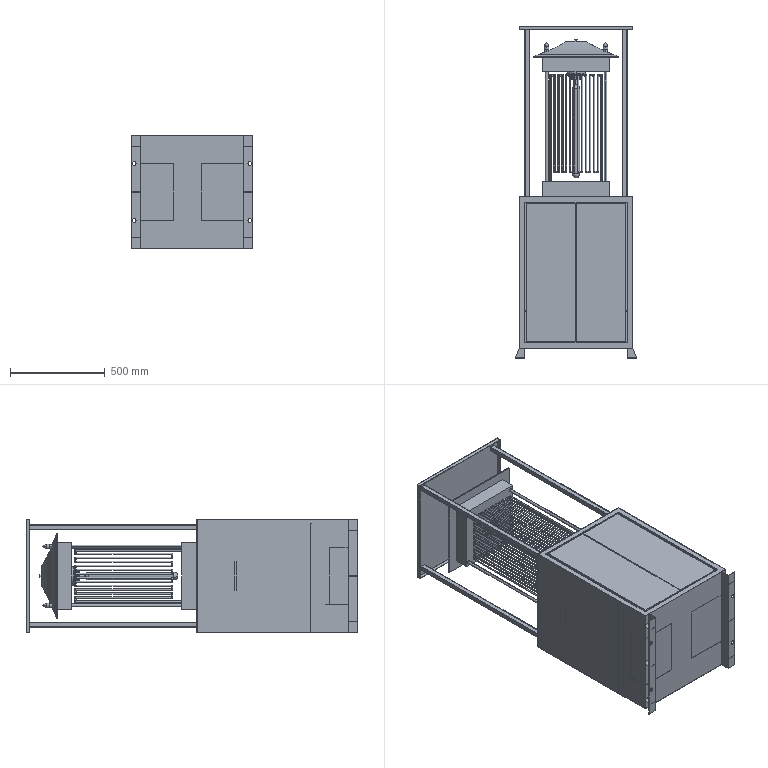Assembly | SolidWorks | mm | 47 component files | 47 solids | 2764 faces | box 640 x 1750 x 600 mm | volume 31033976 mm3 | cylinder 1488 | plane 1206 | torus 40 | spline 26 | sphere 4 | commonest cylinder face diameters 1 x1001 7 x210 5 x88 2.8 x31 20 x28 15 x26 6 x16 8 x14
Bill of materials:
AwningSupportRod | 4 |  | Long straight hollow tube with a square cross-section and thin walls.
AwningTopPlate | 1 |  | Thin, flat, square plate with no visible features.
Box | 1 |  | Rectangular box made of thin walls with an open top. It has flanges on the vertical front edges with small holes, a rectangular cutout in one wall, small triangular tabs along one edge, and angled foot-like tabs at the bottom.
Brush | 3 |  | Long strip with a raised rectangular rib along one edge and a row of many fine, closely spaced bristles or teeth along the other edge, like a comb.
CabinetDoor | 2 |  | Thin rectangular flat plate with small holes near the ends of its long edges and small square openings visible in the end edge view.
Camera | 1 |  | Square block body with a stepped cylindrical boss and a small side pin on one face. A rectangular arm extends from the block and ends in a flat circular disc.
CameraFillLightBracketTable | 1 |  | Rectangular plate of moderate thickness with a small chamfer or bevel along one edge.
FillLight | 1 |  | Flat annular ring with a thin rectangular tab extending outward from its outer edge.
Funnel | 1 |  | Square pyramid-shaped funnel or horn with a square rim at the wide end. It narrows to a rectangular throat block, which carries a short cylindrical tube stub and an angled side tab.
InfraredProcessingChamber | 1 |  | Thin sheet bent into a U or C-channel shape: two parallel flat faces joined by one back face. One face has a square cutout.
InsectCollectionBox | 1 |  | Solid rectangular block with no visible holes or features.
InsectCollectionPlatform | 1 |  | Thin flat plate with a large rectangular notch cut in from one edge, one round hole, two small square holes, and small raised tab or lug features near one edge.
BracketRod | 4 |  | Straight, slender solid cylindrical rod with flat ends.
ElectricNet | 1 |  | Continuous round-section tube or wire bent into a multi-pass serpentine with many parallel straight runs joined by tight U-bends, filling a rectangular box-shaped envelope, with two straight free ends.
InsectTrapLampBase | 1 |  | Square plate of moderate thickness with one large central circular through hole.
InsectTrapLampTop | 1 |  | Composite square body: a thin square flange plate with a rectangular block on one side. The block face carries four small corner holes and a central stepped concentric circular boss with a small central hole. The opposite side of the flange has a flared, curved-profile taper ending in a smaller flat face with protruding cylindrical pins.
LampTube | 1 |  | Elongated capsule-shaped cylindrical body with hemispherical or rounded ends, and a much thinner coaxial rod or wire extending from one end.
LeftPlatform | 1 |  | Thin square sheet or plate with a narrow short lip bent at about 90 degrees along one edge, giving a shallow L-shaped section.
Pin | 4 |  | Solid flanged cylinder: a cylindrical body standing on a larger-diameter thin circular flange whose outer bottom edge is rounded.
PushRod | 1 |  | Straight, slender solid cylindrical rod with flat ends.
PushRodCylinder | 1 |  | Thick-walled cylindrical sleeve, longer than its diameter, with a small coaxial bore.
PushRodFixingRing | 2 |  | Short thin-walled ring or band with a large central opening, with one outer circumferential edge rounded.
SlideRailSupport | 2 |  | Rectangular block with one rounded long edge and two round holes on perpendicular axes: one in the top face and one in a side face.
SlideRod | 2 |  | Very slender straight solid cylindrical rod or wire with flat ends.
SlideTablePlatform | 1 |  | Thin rectangular plate with raised rectangular pads/blocks at both ends of one face, positioned near the corners, with small holes through the blocks and edge.
TopCover | 4 |  | Axisymmetric cap: a hollow cylindrical sleeve that steps down into a closed, domed end with a turned stepped/bulbous profile.
WaterCollectionBox | 1 |  | Plain solid rectangular block (cuboid) with no visible features.
WaterPipe | 1 |  | Hollow round tube bent along a 3D path with several bends, open at both ends.
WireBox | 1 |  | Rectangular box-shaped enclosure or body with chamfered edges, with several rectangular openings on one narrow end face.
Mates:
1. coincident | Box-1 face at (298.5, 800, -300) dir (-1, 0, 0) | InfraredProcessingChamber-1 face at (298.5, 270, 0) dir (1, 0, 0)
2. coincident | Box-1 plane at (0, 0, 0) dir (0, 0, 1) | InfraredProcessingChamber-1 plane at (175, 270, 0) dir (0, 0, 1)
3. coincident | Box-1 face at (0, 1.5, 0) dir (0, 1, 0) | InsectCollectionBox-1 face at (173.5, 1.5, 0) dir (0, -1, 0)
4. coincident | Box-1 face at (298.5, 800, -300) dir (-1, 0, 0) | InsectCollectionBox-1 face at (298.5, 101.5, 150) dir (1, 0, 0)
5. coincident | Box-1 plane at (0, 0, 0) dir (0, 0, 1) | InsectCollectionBox-1 plane at (173.5, 1.5, 0) dir (0, 0, -1)
6. coincident | AwningTopPlate-1 plane at (0, 1680, 0) dir (0, 0, 1) | assembly plane at (0, 0, 0) dir (0, 0, 1)
7. coincident | AwningTopPlate-1 plane at (0, 1680, 0) dir (1, 0, 0) | assembly plane at (0, 0, 0) dir (1, 0, 0)
8. coincident | Box-1 face at (-298.5, 800, -300) dir (1, 0, 0) | InsectCollectionPlatform-1 face at (-298.5, 200, -10) dir (-1, 0, 0)
9. coincident | Box-1 face at (-300, 800, -298.5) dir (0, 0, 1) | InsectCollectionPlatform-1 face at (0, 200, -298.5) dir (0, 0, -1)
10. distance | InfraredProcessingChamber-1 face at (175, 270, 0) dir (0, -1, 0) | InsectCollectionPlatform-1 face at (0, 200, -10) dir (0, 1, 0)
11. distance | InsectCollectionPlatform-1 face at (0, 200, -10) dir (0, 1, 0) | Box-1 face at (0, 800, 0) dir (0, 1, 0)
12. coincident | AwningSupportRod-1 face at (-257.5, 1698.5, 257.5) dir (0, 1, 0) | AwningTopPlate-1 face at (0, 1698.5, 0) dir (0, -1, 0)
13. coincident | Box-1 face at (0, 800, 0) dir (0, 1, 0) | AwningSupportRod-1 face at (-257.5, 800, 257.5) dir (0, -1, 0)
14. parallel | AwningSupportRod-1 face at (-270, 1698.5, 245) dir (-1, 0, 0) | AwningSupportRod-3 face at (-270, 1698.5, -245) dir (-1, 0, 0)
15. parallel | AwningSupportRod-1 face at (-270, 1698.5, 270) dir (0, 0, 1) | AwningSupportRod-3 face at (-245, 1698.5, -245) dir (0, 0, 1)
16. coincident | AwningSupportRod-3 face at (-257.5, 1698.5, -257.5) dir (0, 1, 0) | AwningTopPlate-1 face at (0, 1698.5, 0) dir (0, -1, 0)
17. coincident | AwningSupportRod-7 face at (257.5, 1698.5, 257.5) dir (0, 1, 0) | AwningTopPlate-1 face at (0, 1698.5, 0) dir (0, -1, 0)
18. coincident | AwningSupportRod-5 face at (257.5, 1698.5, -257.5) dir (0, 1, 0) | AwningTopPlate-1 face at (0, 1698.5, 0) dir (0, -1, 0)
19. distance | CabinetDoor-1 face at (-132, 400, 290) dir (0, 0, -1) | Box-1 face at (0, 0, 280) dir (0, 0, 1)
20. distance | CabinetDoor-1 face at (-260, 400, 300) dir (-1, 0, 0) | Box-1 face at (-270, 770, 298.5) dir (1, 0, 0)
21. distance | Box-1 face at (-270, 770, 298.5) dir (0, -1, 0) | CabinetDoor-1 face at (-132, 766, 300) dir (0, 1, 0)
22. coincident | Box-1 face at (-300, 800, 300) dir (0, 0, 1) | CabinetDoor-2 face at (129, 400, 300) dir (0, 0, 1)
23. distance | CabinetDoor-2 face at (260, 400, 300) dir (1, 0, 0) | Box-1 face at (270, 770, 298.5) dir (-1, 0, 0)
24. distance | Box-1 face at (-270, 770, 298.5) dir (0, -1, 0) | CabinetDoor-2 face at (129, 766, 300) dir (0, 1, 0)
25. symmetric | AwningSupportRod-5 face at (270, 1698.5, -245) dir (0, 0, 1) | AwningSupportRod-7 face at (270, 1698.5, 245) dir (0, 0, -1) | assembly plane at (0, 0, 0) dir (0, 0, 1)
26. symmetric | AwningSupportRod-1 face at (-270, 1698.5, 245) dir (0, 0, -1) | AwningSupportRod-3 face at (-245, 1698.5, -245) dir (0, 0, 1) | assembly plane at (0, 0, 0) dir (0, 0, 1)
27. symmetric | AwningSupportRod-1 face at (-245, 1698.5, 245) dir (1, 0, 0) | AwningSupportRod-7 face at (245, 1698.5, 270) dir (-1, 0, 0) | assembly plane at (0, 0, 0) dir (1, 0, 0)
28. symmetric | AwningSupportRod-3 face at (-245, 1698.5, -245) dir (1, 0, 0) | AwningSupportRod-5 face at (245, 1698.5, -245) dir (-1, 0, 0) | assembly plane at (0, 0, 0) dir (1, 0, 0)
29. coincident | AwningSupportRod-1 face at (-270, 1698.5, 245) dir (-1, 0, 0) | AwningSupportRod-3 face at (-270, 1698.5, -245) dir (-1, 0, 0)
30. coincident | AwningSupportRod-1 face at (-270, 1698.5, 270) dir (0, 0, 1) | AwningSupportRod-7 face at (270, 1698.5, 270) dir (0, 0, 1)
31. distance | AwningSupportRod-7 face at (270, 1698.5, 270) dir (0, 0, 1) | Box-1 face at (-300, 800, 300) dir (0, 0, 1)
32. distance | AwningSupportRod-7 face at (270, 1698.5, 270) dir (1, 0, 0) | Box-1 face at (300, 800, -300) dir (1, 0, 0)
33. coincident | Box-1 face at (-298.5, 800, -300) dir (1, 0, 0) | LeftPlatform-1 face at (-298.5, 598.5, -75) dir (-1, 0, 0)
34. distance | LeftPlatform-1 face at (-223.5, 598.5, 0) dir (0, 1, 0) | Box-1 face at (0, 798.5, 0) dir (0, -1, 0)
35. coincident | LeftPlatform-1 plane at (-223.5, 597, 0) dir (0, 0, 1) | assembly plane at (0, 0, 0) dir (0, 0, 1)
36. coincident | Box-1 face at (0, 1.5, 0) dir (0, 1, 0) | WaterCollectionBox-1 face at (-198.5, 1.5, 0) dir (0, -1, 0)
37. coincident | Box-1 face at (-198.5, 1.5, -150) dir (0, 0, 1) | WaterCollectionBox-1 face at (-298.5, 101.5, -150) dir (0, 0, -1)
38. coincident | Box-1 face at (-298.5, 800, -300) dir (1, 0, 0) | WaterCollectionBox-1 face at (-298.5, 101.5, -150) dir (-1, 0, 0)
39. coincident | Box-1 face at (0, 798.5, 0) dir (0, -1, 0) | Funnel-1 face at (0, 798.5, 0) dir (0, 1, 0)
40. coincident | Funnel-1 plane at (0, 798.5, 0) dir (0, 0, 1) | assembly plane at (0, 0, 0) dir (0, 0, 1)
41. coincident | Funnel-1 plane at (0, 798.5, 0) dir (1, 0, 0) | assembly plane at (0, 0, 0) dir (1, 0, 0)
42. parallel | Box-1 face at (-300, 800, 300) dir (0, 0, 1) | InsectTrapLamp-1/InsectTrapLampBase-1 face at (-175, 760, 175) dir (0, 0, 1)
43. concentric | Funnel-1 face at (0, 498.5, 0) dir (0, -1, 0) r 14.5 | WaterPipe-1 face at (0, 402.999, 0) dir (0, 1, 0) r 16
44. coincident | Funnel-1 face at (0, 447, 0) dir (0, -1, 0) | WaterPipe-1 face at (0, 447, 0) dir (0, 1, 0)
45. concentric | InsectCollectionPlatform-1 face at (-248.5, 198.5, -10) dir (0, 1, 0) r 20 | WaterPipe-1 face at (-248.5, 120, -10) dir (0, 1, 0) r 17.5
46. coincident | InfraredProcessingChamber-1 face at (300, 571, 125) dir (0, 0, 1) | Brush-1 face at (48.5, 270, 125) dir (0, 0, -1)
47. coincident | InfraredProcessingChamber-1 face at (175, 270, 0) dir (0, -1, 0) | Brush-1 face at (48.5, 270, 135) dir (0, -1, 0)
48. coincident | Box-1 face at (298.5, 800, -300) dir (-1, 0, 0) | Brush-1 face at (298.5, 270, 125) dir (1, 0, 0)
49. coincident | InfraredProcessingChamber-1 face at (50, 571, -125) dir (-1, 0, 0) | Brush-3 face at (50, 270, -125) dir (1, 0, 0)
50. coincident | InfraredProcessingChamber-1 face at (300, 571, 125) dir (0, 0, 1) | Brush-3 face at (50, 270, 125) dir (0, 0, 1)
51. coincident | InfraredProcessingChamber-1 face at (175, 270, 0) dir (0, -1, 0) | Brush-3 face at (40, 270, -125) dir (0, -1, 0)
52. coincident | InfraredProcessingChamber-1 face at (300, 571, -125) dir (0, 0, -1) | Brush-2 face at (298.5, 270, -125) dir (0, 0, 1)
53. coincident | Box-1 face at (298.5, 800, -300) dir (-1, 0, 0) | Brush-2 face at (298.5, 270, -125) dir (1, 0, 0)
54. coincident | InfraredProcessingChamber-1 face at (175, 270, 0) dir (0, -1, 0) | Brush-2 face at (298.5, 270, -135) dir (0, -1, 0)
55. coincident | InsectCollectionPlatform-1 face at (-184, 195, -10) dir (-1, 0, 0) | SlideRailSupport-1 face at (-184, 198.5, 132.5) dir (1, 0, 0)
56. coincident | InsectCollectionPlatform-1 face at (0, 198.5, -10) dir (0, -1, 0) | SlideRailSupport-1 face at (-191.5, 198.5, 125) dir (0, -1, 0)
57. coincident | InsectCollectionPlatform-1 face at (0, 195, 117.5) dir (0, 0, 1) | SlideRailSupport-1 face at (-199, 198.5, 117.5) dir (0, 0, -1)
58. concentric | SlideRailSupport-1 face at (-195, 220, 125) dir (1, 0, 0) r 2.5 | SlideRod-1 face at (298.5, 220, 125) dir (-1, 0, 0) r 2.5
59. coincident | SlideRailSupport-1 face at (-195, 220, 125) dir (1, 0, 0) | SlideRod-1 face at (-195, 220, 125) dir (-1, 0, 0)
60. coincident | InsectCollectionPlatform-1 face at (-199, 195, -10) dir (1, 0, 0) | SlideRailSupport-2 face at (-199, 198.5, -137.5) dir (-1, 0, 0)
61. coincident | InsectCollectionPlatform-1 face at (0, 198.5, -10) dir (0, -1, 0) | SlideRailSupport-2 face at (-191.5, 198.5, -145) dir (0, -1, 0)
62. coincident | InsectCollectionPlatform-1 face at (0, 195, -152.5) dir (0, 0, 1) | SlideRailSupport-2 face at (-199, 198.5, -152.5) dir (0, 0, -1)
63. concentric | SlideRailSupport-2 face at (-195, 220, -145) dir (1, 0, 0) r 2.5 | SlideRod-2 face at (298.5, 220, -145) dir (-1, 0, 0) r 2.5
64. coincident | SlideRailSupport-2 face at (-195, 220, -145) dir (1, 0, 0) | SlideRod-2 face at (-195, 220, -145) dir (-1, 0, 0)
65. concentric | SlideRod-2 face at (298.5, 220, -145) dir (-1, 0, 0) r 2.5 | SlideTablePlatform-1 face at (32.663, 220, -145) dir (1, 0, 0) r 2.5
66. concentric | SlideRod-1 face at (298.5, 220, 125) dir (-1, 0, 0) r 2.5 | SlideTablePlatform-1 face at (32.663, 220, 125) dir (1, 0, 0) r 2.5
67. coincident | InsectCollectionPlatform-1 face at (-219.5, 205, -20.5) dir (1, 0, 0) | PushRodCylinder-1 face at (-219.5, 220, -10) dir (-1, 0, 0)
68. concentric | InsectCollectionPlatform-1 face at (-183.5, 220, -10) dir (1, 0, 0) r 4 | PushRodCylinder-1 face at (-203.5, 220, -10) dir (1, 0, 0) r 4
69. concentric | PushRodCylinder-1 face at (-203.5, 220, -10) dir (1, 0, 0) r 4 | PushRod-1 face at (96.5, 220, -10) dir (-1, 0, 0) r 4
70. coincident | PushRodCylinder-1 face at (-203.5, 220, -10) dir (1, 0, 0) | PushRod-1 face at (-203.5, 220, -10) dir (-1, 0, 0)
71. coincident | SlideTablePlatform-1 face at (32.663, 230.5, 130) dir (-1, 0, 0) | PushRodFixingRing-1 face at (32.663, 220, -10) dir (1, 0, 0)
72. concentric | PushRod-1 face at (96.5, 220, -10) dir (-1, 0, 0) r 4 | PushRodFixingRing-1 face at (29.663, 220, -10) dir (1, 0, 0) r 4
73. concentric | PushRod-1 face at (96.5, 220, -10) dir (-1, 0, 0) r 4 | PushRodFixingRing-2 face at (37.663, 220, -10) dir (-1, 0, 0) r 4
74. coincident | SlideTablePlatform-1 face at (34.663, -47.508, 120) dir (1, 0, 0) | PushRodFixingRing-2 face at (34.663, 220, -10) dir (-1, 0, 0)
75. distance | SlideTablePlatform-1 face at (32.663, 230.5, 130) dir (-1, 0, 0) | SlideRailSupport-1 face at (-184, 198.5, 132.5) dir (1, 0, 0)
76. concentric | SlideRailSupport-1 face at (-191.5, 220, 107.5) dir (0, 0, 1) r 2.5 | Pin-4 face at (-191.5, 220, 132.5) dir (0, 0, -1) r 2.5
77. coincident | SlideRailSupport-1 face at (-199, 198.5, 132.5) dir (0, 0, 1) | Pin-4 face at (-191.5, 220, 132.5) dir (0, 0, -1)
78. concentric | SlideRailSupport-1 face at (-191.5, 220, 107.5) dir (0, 0, 1) r 2.5 | Pin-1 face at (-191.5, 220, 117.5) dir (0, 0, 1) r 2.5
79. coincident | SlideRailSupport-1 face at (-199, 198.5, 117.5) dir (0, 0, -1) | Pin-1 face at (-191.5, 220, 117.5) dir (0, 0, 1)
80. concentric | SlideRailSupport-2 face at (-191.5, 220, -162.5) dir (0, 0, 1) r 2.5 | Pin-3 face at (-191.5, 220, -152.5) dir (0, 0, 1) r 2.5
81. coincident | SlideRailSupport-2 face at (-199, 198.5, -152.5) dir (0, 0, -1) | Pin-3 face at (-191.5, 220, -152.5) dir (0, 0, 1)
82. concentric | SlideRailSupport-2 face at (-191.5, 220, -162.5) dir (0, 0, 1) r 2.5 | Pin-2 face at (-191.5, 220, -137.5) dir (0, 0, -1) r 2.5
83. coincident | SlideRailSupport-2 face at (-199, 198.5, -137.5) dir (0, 0, 1) | Pin-2 face at (-191.5, 220, -137.5) dir (0, 0, -1)
84. concentric | InsectTrapLamp-1/InsectTrapLampTop-1 face at (-155, 1590, -155) dir (0, -1, 0) r 10 | TopCover-2 face at (-155, 1592.5, -155) dir (0, -1, 0) r 10
85. coincident | InsectTrapLamp-1/InsectTrapLampTop-1 face at (0, 1590, 0) dir (0, 1, 0) | TopCover-2 face at (-155, 1590, -155) dir (0, -1, 0)
86. concentric | InsectTrapLamp-1/InsectTrapLampTop-1 face at (-155, 1590, 155) dir (0, -1, 0) r 10 | TopCover-4 face at (-155, 1592.5, 155) dir (0, -1, 0) r 10
87. concentric | InsectTrapLamp-1/InsectTrapLampTop-1 face at (155, 1590, 155) dir (0, -1, 0) r 10 | TopCover-3 face at (155, 1592.5, 155) dir (0, -1, 0) r 10
88. concentric | InsectTrapLamp-1/InsectTrapLampTop-1 face at (155, 1590, -155) dir (0, -1, 0) r 10 | TopCover-1 face at (155, 1592.5, -155) dir (0, -1, 0) r 10
89. coincident | TopCover-1 face at (155, 1577.5, -155) dir (0, -1, 0) | TopCover-2 face at (-155, 1577.5, -155) dir (0, -1, 0)
90. coincident | TopCover-2 face at (-155, 1577.5, -155) dir (0, -1, 0) | TopCover-4 face at (-155, 1577.5, 155) dir (0, -1, 0)
91. coincident | TopCover-3 face at (155, 1577.5, 155) dir (0, -1, 0) | TopCover-4 face at (-155, 1577.5, 155) dir (0, -1, 0)
92. coincident | Box-1 face at (0, 800, 0) dir (0, 1, 0) | InsectTrapLamp-1/InsectTrapLampBase-1 face at (0, 800, 0) dir (0, -1, 0)
93. concentric | Funnel-1 face at (0, 498.5, 0) dir (0, -1, 0) r 16 | InsectTrapLamp-1/InsectTrapLampBase-1 face at (0, 802, 0) dir (0, -1, 0) r 75
94. coincident | Box-1 face at (298.5, 800, -300) dir (-1, 0, 0) | CameraFillLightBracketTable-1 face at (298.5, 600, 0) dir (1, 0, 0)
95. concentric | CameraFillLightBracketTable-1 face at (295.5, 600, 0) dir (-1, 0, 0) r 15 | Camera-1 face at (289.5, 600, 0) dir (1, 0, 0) r 15
96. coincident | Box-1 face at (295.5, 630, -50) dir (0, -1, 0) | CameraFillLightBracketTable-1 face at (293.5, 630, -50) dir (0, 1, 0)
97. coincident | Box-1 face at (295.5, 630, -50) dir (0, 0, 1) | CameraFillLightBracketTable-1 face at (293.5, 630, -50) dir (0, 0, -1)
98. coincident | CameraFillLightBracketTable-1 face at (295.5, 600, 0) dir (-1, 0, 0) | Camera-1 face at (295.5, 600, 0) dir (1, 0, 0)
99. coincident | CameraFillLightBracketTable-1 face at (295.5, 600, 0) dir (-1, 0, 0) | FillLight-1 face at (295.5, 579, 0) dir (1, 0, 0)
100. coincident | CameraFillLightBracketTable-1 face at (295.5, 581.5, -6) dir (0, 0, 1) | FillLight-1 face at (175.5, 581.5, -6) dir (0, 0, -1)
101. coincident | CameraFillLightBracketTable-1 edge at (293.5, 581.5, 6) dir (0, 0, -1) | FillLight-1 face at (175.5, 581.5, -6) dir (0, 1, 0)
102. coincident | LeftPlatform-1 face at (-223.5, 598.5, 0) dir (0, 1, 0) | WireBox-1 face at (-213.5, 598.5, 5) dir (0, -1, 0)
103. distance | LeftPlatform-1 face at (-298.5, 598.5, 75) dir (0, 0, 1) | WireBox-1 face at (-183.5, 618.5, 55) dir (0, 0, 1)
104. distance | Box-1 face at (-298.5, 800, -300) dir (1, 0, 0) | WireBox-1 face at (-248.5, 618.5, -40) dir (-1, 0, 0)
105. coincident | InsectTrapLampBase-1 face at (-172.45, -14.429, 575) dir (0, 0, 1) | InsectTrapLampTop-1 face at (-172.45, 765.571, 575) dir (0, 0, 1)
106. coincident | InsectTrapLampBase-1 face at (-172.45, -14.429, 225) dir (-1, 0, 0) | InsectTrapLampTop-1 face at (-172.45, 765.571, 225) dir (-1, 0, 0)
107. concentric | InsectTrapLampTop-1 face at (2.55, 685.571, 400) dir (0, 1, 0) r 5 | LampTube-1 face at (2.55, 855.571, 400) dir (0, -1, 0) r 5
108. coincident | InsectTrapLampTop-1 face at (2.55, 855.571, 400) dir (0, 1, 0) | LampTube-1 face at (2.55, 855.571, 400) dir (0, 1, 0)
109. concentric | InsectTrapLampBase-1 face at (-132.45, 95.571, 535) dir (0, 1, 0) r 2.5 | ElectricNet-1 face at (-132.45, 105.572, 535) dir (0, 1, 0) r 3.5
110. concentric | InsectTrapLampBase-1 face at (-152.45, 85.571, 555) dir (0, 1, 0) r 7.5 | BracketRod-5 face at (-152.45, 815.571, 555) dir (0, -1, 0) r 7.5
111. coincident | InsectTrapLampBase-1 face at (-152.45, 85.571, 555) dir (0, 1, 0) | BracketRod-5 face at (-152.45, 85.571, 555) dir (0, -1, 0)
112. coincident | InsectTrapLampTop-1 face at (2.55, 815.571, 400) dir (0, 1, 0) | BracketRod-5 face at (-152.45, 815.571, 555) dir (0, 1, 0)
113. concentric | InsectTrapLampBase-1 face at (157.55, 85.571, 555) dir (0, 1, 0) r 7.5 | BracketRod-8 face at (157.55, 815.571, 555) dir (0, -1, 0) r 7.5
114. concentric | InsectTrapLampBase-1 face at (157.55, 85.571, 245) dir (0, 1, 0) r 7.5 | BracketRod-7 face at (157.55, 815.571, 245) dir (0, -1, 0) r 7.5
115. concentric | InsectTrapLampBase-1 face at (-152.45, 85.571, 245) dir (0, 1, 0) r 7.5 | BracketRod-6 face at (-152.45, 815.571, 245) dir (0, -1, 0) r 7.5
116. coincident | InsectTrapLampTop-1 face at (2.55, 815.571, 400) dir (0, 1, 0) | BracketRod-6 face at (-152.45, 815.571, 245) dir (0, 1, 0)
117. coincident | InsectTrapLampTop-1 face at (2.55, 815.571, 400) dir (0, 1, 0) | BracketRod-7 face at (157.55, 815.571, 245) dir (0, 1, 0)
118. coincident | InsectTrapLampTop-1 face at (2.55, 815.571, 400) dir (0, 1, 0) | BracketRod-8 face at (157.55, 815.571, 555) dir (0, 1, 0)